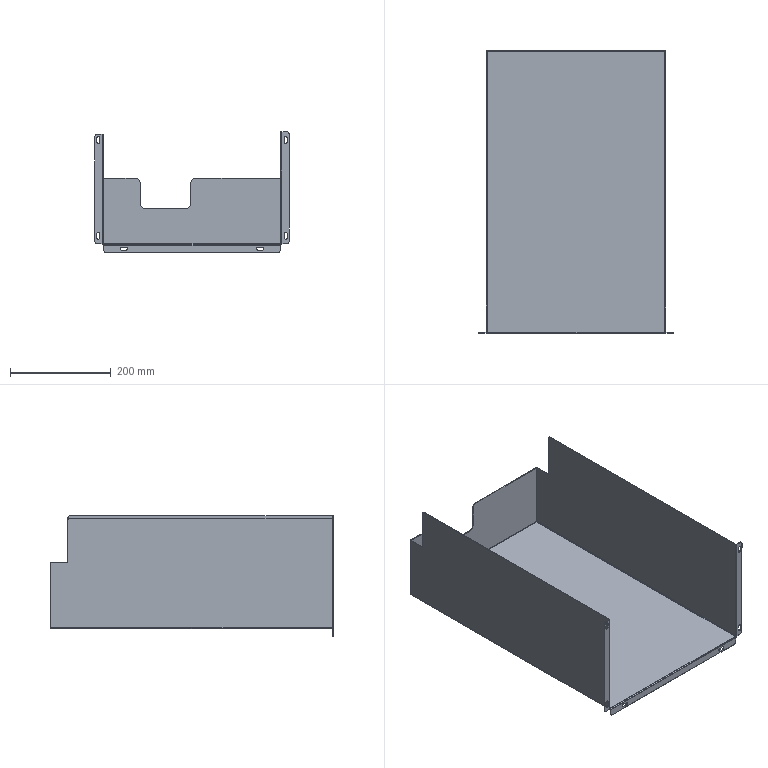Component | SolidWorks | -TractorCover-2 | 1 solid | 106 faces | volume 732456 mm3 | plane 68 | cylinder 38 | commonest cylinder face diameters 6 x14 10 x8 4.473 x6 1.473 x6 20 x4